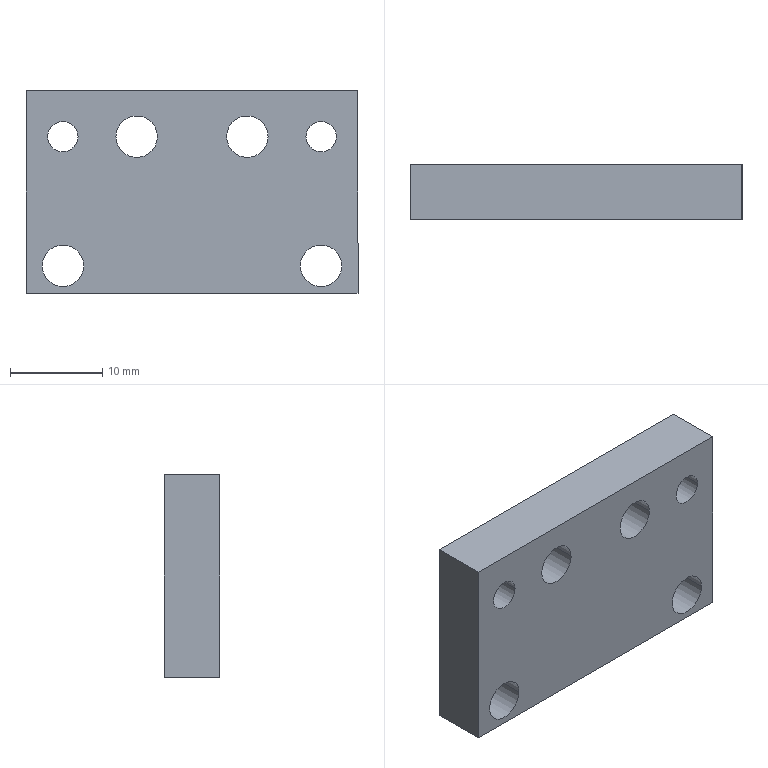Component | SolidWorks | AdjustingPlate-1 | 1 solid | 18 faces | box 36 x 6 x 22 mm | volume 4268 mm3 | cylinder 12 | plane 6 | commonest cylinder face diameters 4.5 x8 3.3 x4
build123d program:
from build123d import *

# Parameters (mm, degrees)
SKETCH1_W                      = 36
SKETCH1_H                      = 22
EXTRUDE1_DEPTH                 = 6
F_4_5_4_5_DIAMETER_HOLE1_D     = 4.5
F_4_5_4_5_DIAMETER_HOLE1_DEPTH = 6.5
F_4_5_4_5_DIAMETER_HOLE1_TIP   = 1.352
SKETCH4_R                      = 2.25
EXTRUDE2_DEPTH                 = 22.932
M4_TAPPED_HOLE1_D              = 3.3
M4_TAPPED_HOLE1_DEPTH          = 11.5
M4_TAPPED_HOLE1_TIP            = 0.9914


with BuildPart() as part:
    # Sketch1 → Extrude1 (new body)
    with BuildSketch(Plane.XY):
        Rectangle(SKETCH1_W, SKETCH1_H)
    extrude(amount=EXTRUDE1_DEPTH)

    # 4.5 _4.5_ Diameter Hole1
    with Locations(Plane.XY.offset(6)):
        with Locations((-14, -8), (14, -8)):
            Hole(F_4_5_4_5_DIAMETER_HOLE1_D / 2, depth=F_4_5_4_5_DIAMETER_HOLE1_DEPTH)
            with Locations((0, 0, -(F_4_5_4_5_DIAMETER_HOLE1_DEPTH + F_4_5_4_5_DIAMETER_HOLE1_TIP / 2))):  # 118° drill point
                Cone(0, F_4_5_4_5_DIAMETER_HOLE1_D / 2, F_4_5_4_5_DIAMETER_HOLE1_TIP, mode=Mode.SUBTRACT)

    # Sketch4 → Extrude2 (cut, through all)
    with BuildSketch(Plane.XY.offset(6)):
        with Locations((-6, 6)):
            Circle(SKETCH4_R)
        with Locations((6, 6)):
            Circle(SKETCH4_R)
    extrude(amount=-EXTRUDE2_DEPTH, mode=Mode.SUBTRACT)

    # M4 Tapped Hole1
    with Locations(Plane.XY.offset(6)):
        with Locations((-14, 6), (14, 6)):
            Hole(M4_TAPPED_HOLE1_D / 2, depth=M4_TAPPED_HOLE1_DEPTH)
            with Locations((0, 0, -(M4_TAPPED_HOLE1_DEPTH + M4_TAPPED_HOLE1_TIP / 2))):  # 118° drill point
                Cone(0, M4_TAPPED_HOLE1_D / 2, M4_TAPPED_HOLE1_TIP, mode=Mode.SUBTRACT)


solid = part.part

# Placed as in the assembly
solid = solid.moved(Location((-50, 166.5, -159.197), (90, 0, 0)))
STEP:
#1=COLOUR_RGB('',0.7922,0.8196,0.9333);
#2=FILL_AREA_STYLE_COLOUR('',#1);
#3=FILL_AREA_STYLE('',(#2));
#4=SURFACE_STYLE_FILL_AREA(#3);
#5=SURFACE_SIDE_STYLE('',(#4));
#6=SURFACE_STYLE_USAGE(.BOTH.,#5);
#7=PRESENTATION_STYLE_ASSIGNMENT((#6));
#8=CARTESIAN_POINT('',(-2.585,6.555,-6.031));
#9=VERTEX_POINT('',#8);
#10=CARTESIAN_POINT('',(-2.455,6.555,-6.031));
#11=VERTEX_POINT('',#10);
#12=CARTESIAN_POINT('',(-2.52,6.555,-6.031));
#13=DIRECTION('',(-0.,-1.,0.));
#14=DIRECTION('',(1.,0.,0.));
#15=AXIS2_PLACEMENT_3D('',#12,#13,#14);
#16=CIRCLE('',#15,0.06496);
#17=EDGE_CURVE('',#9,#11,#16,.T.);
#18=ORIENTED_EDGE('',*,*,#17,.F.);
#19=CARTESIAN_POINT('',(-2.585,6.319,-6.031));
#20=VERTEX_POINT('',#19);
#21=CARTESIAN_POINT('',(-2.585,6.319,-6.031));
#22=DIRECTION('',(-0.,-1.,0.));
#23=VECTOR('',#22,39.37);
#24=LINE('',#21,#23);
#25=EDGE_CURVE('',#9,#20,#24,.T.);
#26=ORIENTED_EDGE('',*,*,#25,.T.);
#27=CARTESIAN_POINT('',(-2.455,6.319,-6.031));
#28=VERTEX_POINT('',#27);
#29=CARTESIAN_POINT('',(-2.52,6.319,-6.031));
#30=DIRECTION('',(-0.,-1.,0.));
#31=DIRECTION('',(1.,0.,0.));
#32=AXIS2_PLACEMENT_3D('',#29,#30,#31);
#33=CIRCLE('',#32,0.06496);
#34=EDGE_CURVE('',#20,#28,#33,.T.);
#35=ORIENTED_EDGE('',*,*,#34,.T.);
#36=CARTESIAN_POINT('',(-2.455,6.319,-6.031));
#37=DIRECTION('',(-0.,-1.,0.));
#38=VECTOR('',#37,39.37);
#39=LINE('',#36,#38);
#40=EDGE_CURVE('',#11,#28,#39,.T.);
#41=ORIENTED_EDGE('',*,*,#40,.F.);
#42=EDGE_LOOP('',(#18,#26,#35,#41));
#43=FACE_OUTER_BOUND('',#42,.T.);
#44=CARTESIAN_POINT('',(-2.52,6.319,-6.031));
#45=DIRECTION('',(-0.,-1.,0.));
#46=DIRECTION('',(1.,0.,0.));
#47=AXIS2_PLACEMENT_3D('',#44,#45,#46);
#48=CYLINDRICAL_SURFACE('',#47,0.06496);
#49=ADVANCED_FACE('',(#43),#48,.F.);
#50=CARTESIAN_POINT('',(-1.482,6.555,-6.031));
#51=VERTEX_POINT('',#50);
#52=CARTESIAN_POINT('',(-1.352,6.555,-6.031));
#53=VERTEX_POINT('',#52);
#54=CARTESIAN_POINT('',(-1.417,6.555,-6.031));
#55=DIRECTION('',(-0.,-1.,0.));
#56=DIRECTION('',(1.,0.,0.));
#57=AXIS2_PLACEMENT_3D('',#54,#55,#56);
#58=CIRCLE('',#57,0.06496);
#59=EDGE_CURVE('',#51,#53,#58,.T.);
#60=ORIENTED_EDGE('',*,*,#59,.F.);
#61=CARTESIAN_POINT('',(-1.482,6.319,-6.031));
#62=VERTEX_POINT('',#61);
#63=CARTESIAN_POINT('',(-1.482,6.319,-6.031));
#64=DIRECTION('',(-0.,-1.,0.));
#65=VECTOR('',#64,39.37);
#66=LINE('',#63,#65);
#67=EDGE_CURVE('',#51,#62,#66,.T.);
#68=ORIENTED_EDGE('',*,*,#67,.T.);
#69=CARTESIAN_POINT('',(-1.352,6.319,-6.031));
#70=VERTEX_POINT('',#69);
#71=CARTESIAN_POINT('',(-1.417,6.319,-6.031));
#72=DIRECTION('',(-0.,-1.,0.));
#73=DIRECTION('',(1.,0.,0.));
#74=AXIS2_PLACEMENT_3D('',#71,#72,#73);
#75=CIRCLE('',#74,0.06496);
#76=EDGE_CURVE('',#62,#70,#75,.T.);
#77=ORIENTED_EDGE('',*,*,#76,.T.);
#78=CARTESIAN_POINT('',(-1.352,6.319,-6.031));
#79=DIRECTION('',(-0.,-1.,0.));
#80=VECTOR('',#79,39.37);
#81=LINE('',#78,#80);
#82=EDGE_CURVE('',#53,#70,#81,.T.);
#83=ORIENTED_EDGE('',*,*,#82,.F.);
#84=EDGE_LOOP('',(#60,#68,#77,#83));
#85=FACE_OUTER_BOUND('',#84,.T.);
#86=CARTESIAN_POINT('',(-1.417,6.319,-6.031));
#87=DIRECTION('',(-0.,-1.,0.));
#88=DIRECTION('',(1.,0.,0.));
#89=AXIS2_PLACEMENT_3D('',#86,#87,#88);
#90=CYLINDRICAL_SURFACE('',#89,0.06496);
#91=ADVANCED_FACE('',(#85),#90,.F.);
#92=CARTESIAN_POINT('',(-1.821,6.555,-6.031));
#93=VERTEX_POINT('',#92);
#94=CARTESIAN_POINT('',(-1.644,6.555,-6.031));
#95=VERTEX_POINT('',#94);
#96=CARTESIAN_POINT('',(-1.732,6.555,-6.031));
#97=DIRECTION('',(-0.,-1.,0.));
#98=DIRECTION('',(1.,0.,0.));
#99=AXIS2_PLACEMENT_3D('',#96,#97,#98);
#100=CIRCLE('',#99,0.08858);
#101=EDGE_CURVE('',#93,#95,#100,.T.);
#102=ORIENTED_EDGE('',*,*,#101,.F.);
#103=CARTESIAN_POINT('',(-1.821,6.319,-6.031));
#104=VERTEX_POINT('',#103);
#105=CARTESIAN_POINT('',(-1.821,6.555,-6.031));
#106=DIRECTION('',(-0.,-1.,0.));
#107=VECTOR('',#106,39.37);
#108=LINE('',#105,#107);
#109=EDGE_CURVE('',#93,#104,#108,.T.);
#110=ORIENTED_EDGE('',*,*,#109,.T.);
#111=CARTESIAN_POINT('',(-1.644,6.319,-6.031));
#112=VERTEX_POINT('',#111);
#113=CARTESIAN_POINT('',(-1.732,6.319,-6.031));
#114=DIRECTION('',(-0.,-1.,0.));
#115=DIRECTION('',(1.,0.,0.));
#116=AXIS2_PLACEMENT_3D('',#113,#114,#115);
#117=CIRCLE('',#116,0.08858);
#118=EDGE_CURVE('',#104,#112,#117,.T.);
#119=ORIENTED_EDGE('',*,*,#118,.T.);
#120=CARTESIAN_POINT('',(-1.644,6.555,-6.031));
#121=DIRECTION('',(-0.,-1.,0.));
#122=VECTOR('',#121,39.37);
#123=LINE('',#120,#122);
#124=EDGE_CURVE('',#95,#112,#123,.T.);
#125=ORIENTED_EDGE('',*,*,#124,.F.);
#126=EDGE_LOOP('',(#102,#110,#119,#125));
#127=FACE_OUTER_BOUND('',#126,.T.);
#128=CARTESIAN_POINT('',(-1.732,6.555,-6.031));
#129=DIRECTION('',(-0.,-1.,0.));
#130=DIRECTION('',(1.,0.,0.));
#131=AXIS2_PLACEMENT_3D('',#128,#129,#130);
#132=CYLINDRICAL_SURFACE('',#131,0.08858);
#133=ADVANCED_FACE('',(#127),#132,.F.);
#134=CARTESIAN_POINT('',(-2.293,6.555,-6.031));
#135=VERTEX_POINT('',#134);
#136=CARTESIAN_POINT('',(-2.116,6.555,-6.031));
#137=VERTEX_POINT('',#136);
#138=CARTESIAN_POINT('',(-2.205,6.555,-6.031));
#139=DIRECTION('',(-0.,-1.,0.));
#140=DIRECTION('',(1.,0.,0.));
#141=AXIS2_PLACEMENT_3D('',#138,#139,#140);
#142=CIRCLE('',#141,0.08858);
#143=EDGE_CURVE('',#135,#137,#142,.T.);
#144=ORIENTED_EDGE('',*,*,#143,.F.);
#145=CARTESIAN_POINT('',(-2.293,6.319,-6.031));
#146=VERTEX_POINT('',#145);
#147=CARTESIAN_POINT('',(-2.293,6.555,-6.031));
#148=DIRECTION('',(-0.,-1.,0.));
#149=VECTOR('',#148,39.37);
#150=LINE('',#147,#149);
#151=EDGE_CURVE('',#135,#146,#150,.T.);
#152=ORIENTED_EDGE('',*,*,#151,.T.);
#153=CARTESIAN_POINT('',(-2.116,6.319,-6.031));
#154=VERTEX_POINT('',#153);
#155=CARTESIAN_POINT('',(-2.205,6.319,-6.031));
#156=DIRECTION('',(-0.,-1.,0.));
#157=DIRECTION('',(1.,0.,0.));
#158=AXIS2_PLACEMENT_3D('',#155,#156,#157);
#159=CIRCLE('',#158,0.08858);
#160=EDGE_CURVE('',#146,#154,#159,.T.);
#161=ORIENTED_EDGE('',*,*,#160,.T.);
#162=CARTESIAN_POINT('',(-2.116,6.555,-6.031));
#163=DIRECTION('',(-0.,-1.,0.));
#164=VECTOR('',#163,39.37);
#165=LINE('',#162,#164);
#166=EDGE_CURVE('',#137,#154,#165,.T.);
#167=ORIENTED_EDGE('',*,*,#166,.F.);
#168=EDGE_LOOP('',(#144,#152,#161,#167));
#169=FACE_OUTER_BOUND('',#168,.T.);
#170=CARTESIAN_POINT('',(-2.205,6.555,-6.031));
#171=DIRECTION('',(-0.,-1.,0.));
#172=DIRECTION('',(1.,0.,0.));
#173=AXIS2_PLACEMENT_3D('',#170,#171,#172);
#174=CYLINDRICAL_SURFACE('',#173,0.08858);
#175=ADVANCED_FACE('',(#169),#174,.F.);
#176=CARTESIAN_POINT('',(-2.608,6.555,-6.583));
#177=VERTEX_POINT('',#176);
#178=CARTESIAN_POINT('',(-2.431,6.555,-6.583));
#179=VERTEX_POINT('',#178);
#180=CARTESIAN_POINT('',(-2.52,6.555,-6.583));
#181=DIRECTION('',(-0.,-1.,0.));
#182=DIRECTION('',(1.,0.,0.));
#183=AXIS2_PLACEMENT_3D('',#180,#181,#182);
#184=CIRCLE('',#183,0.08858);
#185=EDGE_CURVE('',#177,#179,#184,.T.);
#186=ORIENTED_EDGE('',*,*,#185,.F.);
#187=CARTESIAN_POINT('',(-2.608,6.319,-6.583));
#188=VERTEX_POINT('',#187);
#189=CARTESIAN_POINT('',(-2.608,6.319,-6.583));
#190=DIRECTION('',(-0.,-1.,0.));
#191=VECTOR('',#190,39.37);
#192=LINE('',#189,#191);
#193=EDGE_CURVE('',#177,#188,#192,.T.);
#194=ORIENTED_EDGE('',*,*,#193,.T.);
#195=CARTESIAN_POINT('',(-2.431,6.319,-6.583));
#196=VERTEX_POINT('',#195);
#197=CARTESIAN_POINT('',(-2.52,6.319,-6.583));
#198=DIRECTION('',(-0.,-1.,0.));
#199=DIRECTION('',(1.,0.,0.));
#200=AXIS2_PLACEMENT_3D('',#197,#198,#199);
#201=CIRCLE('',#200,0.08858);
#202=EDGE_CURVE('',#188,#196,#201,.T.);
#203=ORIENTED_EDGE('',*,*,#202,.T.);
#204=CARTESIAN_POINT('',(-2.431,6.319,-6.583));
#205=DIRECTION('',(-0.,-1.,0.));
#206=VECTOR('',#205,39.37);
#207=LINE('',#204,#206);
#208=EDGE_CURVE('',#179,#196,#207,.T.);
#209=ORIENTED_EDGE('',*,*,#208,.F.);
#210=EDGE_LOOP('',(#186,#194,#203,#209));
#211=FACE_OUTER_BOUND('',#210,.T.);
#212=CARTESIAN_POINT('',(-2.52,6.319,-6.583));
#213=DIRECTION('',(-0.,-1.,0.));
#214=DIRECTION('',(1.,0.,0.));
#215=AXIS2_PLACEMENT_3D('',#212,#213,#214);
#216=CYLINDRICAL_SURFACE('',#215,0.08858);
#217=ADVANCED_FACE('',(#211),#216,.F.);
#218=CARTESIAN_POINT('',(-1.506,6.555,-6.583));
#219=VERTEX_POINT('',#218);
#220=CARTESIAN_POINT('',(-1.329,6.555,-6.583));
#221=VERTEX_POINT('',#220);
#222=CARTESIAN_POINT('',(-1.417,6.555,-6.583));
#223=DIRECTION('',(-0.,-1.,0.));
#224=DIRECTION('',(1.,0.,0.));
#225=AXIS2_PLACEMENT_3D('',#222,#223,#224);
#226=CIRCLE('',#225,0.08858);
#227=EDGE_CURVE('',#219,#221,#226,.T.);
#228=ORIENTED_EDGE('',*,*,#227,.F.);
#229=CARTESIAN_POINT('',(-1.506,6.319,-6.583));
#230=VERTEX_POINT('',#229);
#231=CARTESIAN_POINT('',(-1.506,6.319,-6.583));
#232=DIRECTION('',(-0.,-1.,0.));
#233=VECTOR('',#232,39.37);
#234=LINE('',#231,#233);
#235=EDGE_CURVE('',#219,#230,#234,.T.);
#236=ORIENTED_EDGE('',*,*,#235,.T.);
#237=CARTESIAN_POINT('',(-1.329,6.319,-6.583));
#238=VERTEX_POINT('',#237);
#239=CARTESIAN_POINT('',(-1.417,6.319,-6.583));
#240=DIRECTION('',(-0.,-1.,0.));
#241=DIRECTION('',(1.,0.,0.));
#242=AXIS2_PLACEMENT_3D('',#239,#240,#241);
#243=CIRCLE('',#242,0.08858);
#244=EDGE_CURVE('',#230,#238,#243,.T.);
#245=ORIENTED_EDGE('',*,*,#244,.T.);
#246=CARTESIAN_POINT('',(-1.329,6.319,-6.583));
#247=DIRECTION('',(-0.,-1.,0.));
#248=VECTOR('',#247,39.37);
#249=LINE('',#246,#248);
#250=EDGE_CURVE('',#221,#238,#249,.T.);
#251=ORIENTED_EDGE('',*,*,#250,.F.);
#252=EDGE_LOOP('',(#228,#236,#245,#251));
#253=FACE_OUTER_BOUND('',#252,.T.);
#254=CARTESIAN_POINT('',(-1.417,6.319,-6.583));
#255=DIRECTION('',(-0.,-1.,0.));
#256=DIRECTION('',(1.,0.,0.));
#257=AXIS2_PLACEMENT_3D('',#254,#255,#256);
#258=CYLINDRICAL_SURFACE('',#257,0.08858);
#259=ADVANCED_FACE('',(#253),#258,.F.);
#260=CARTESIAN_POINT('',(-2.677,6.555,-5.835));
#261=VERTEX_POINT('',#260);
#262=CARTESIAN_POINT('',(-2.677,6.555,-6.701));
#263=VERTEX_POINT('',#262);
#264=CARTESIAN_POINT('',(-2.677,6.555,-6.701));
#265=DIRECTION('',(0.,-0.,-1.));
#266=VECTOR('',#265,39.37);
#267=LINE('',#264,#266);
#268=EDGE_CURVE('',#261,#263,#267,.T.);
#269=ORIENTED_EDGE('',*,*,#268,.T.);
#270=CARTESIAN_POINT('',(-2.677,6.319,-6.701));
#271=VERTEX_POINT('',#270);
#272=CARTESIAN_POINT('',(-2.677,6.319,-6.701));
#273=DIRECTION('',(0.,1.,-0.));
#274=VECTOR('',#273,39.37);
#275=LINE('',#272,#274);
#276=EDGE_CURVE('',#271,#263,#275,.T.);
#277=ORIENTED_EDGE('',*,*,#276,.F.);
#278=CARTESIAN_POINT('',(-2.677,6.319,-5.835));
#279=VERTEX_POINT('',#278);
#280=CARTESIAN_POINT('',(-2.677,6.319,-6.701));
#281=DIRECTION('',(0.,-0.,-1.));
#282=VECTOR('',#281,39.37);
#283=LINE('',#280,#282);
#284=EDGE_CURVE('',#279,#271,#283,.T.);
#285=ORIENTED_EDGE('',*,*,#284,.F.);
#286=CARTESIAN_POINT('',(-2.677,6.319,-5.835));
#287=DIRECTION('',(0.,1.,-0.));
#288=VECTOR('',#287,39.37);
#289=LINE('',#286,#288);
#290=EDGE_CURVE('',#279,#261,#289,.T.);
#291=ORIENTED_EDGE('',*,*,#290,.T.);
#292=EDGE_LOOP('',(#269,#277,#285,#291));
#293=FACE_OUTER_BOUND('',#292,.T.);
#294=CARTESIAN_POINT('',(-2.677,6.319,-6.701));
#295=DIRECTION('',(1.,-0.,0.));
#296=DIRECTION('',(0.,1.,-0.));
#297=AXIS2_PLACEMENT_3D('',#294,#295,#296);
#298=PLANE('',#297);
#299=ADVANCED_FACE('',(#293),#298,.F.);
#300=CARTESIAN_POINT('',(-1.26,6.555,-6.701));
#301=VERTEX_POINT('',#300);
#302=CARTESIAN_POINT('',(-1.26,6.555,-6.701));
#303=DIRECTION('',(1.,-0.,0.));
#304=VECTOR('',#303,39.37);
#305=LINE('',#302,#304);
#306=EDGE_CURVE('',#263,#301,#305,.T.);
#307=ORIENTED_EDGE('',*,*,#306,.T.);
#308=CARTESIAN_POINT('',(-1.26,6.319,-6.701));
#309=VERTEX_POINT('',#308);
#310=CARTESIAN_POINT('',(-1.26,6.319,-6.701));
#311=DIRECTION('',(0.,1.,-0.));
#312=VECTOR('',#311,39.37);
#313=LINE('',#310,#312);
#314=EDGE_CURVE('',#309,#301,#313,.T.);
#315=ORIENTED_EDGE('',*,*,#314,.F.);
#316=CARTESIAN_POINT('',(-1.26,6.319,-6.701));
#317=DIRECTION('',(1.,-0.,0.));
#318=VECTOR('',#317,39.37);
#319=LINE('',#316,#318);
#320=EDGE_CURVE('',#271,#309,#319,.T.);
#321=ORIENTED_EDGE('',*,*,#320,.F.);
#322=ORIENTED_EDGE('',*,*,#276,.T.);
#323=EDGE_LOOP('',(#307,#315,#321,#322));
#324=FACE_OUTER_BOUND('',#323,.T.);
#325=CARTESIAN_POINT('',(-1.26,6.319,-6.701));
#326=DIRECTION('',(-0.,0.,1.));
#327=DIRECTION('',(-1.,0.,-0.));
#328=AXIS2_PLACEMENT_3D('',#325,#326,#327);
#329=PLANE('',#328);
#330=ADVANCED_FACE('',(#324),#329,.F.);
#331=CARTESIAN_POINT('',(-1.26,6.555,-5.835));
#332=VERTEX_POINT('',#331);
#333=CARTESIAN_POINT('',(-1.26,6.555,-6.701));
#334=DIRECTION('',(-0.,0.,1.));
#335=VECTOR('',#334,39.37);
#336=LINE('',#333,#335);
#337=EDGE_CURVE('',#301,#332,#336,.T.);
#338=ORIENTED_EDGE('',*,*,#337,.T.);
#339=CARTESIAN_POINT('',(-1.26,6.319,-5.835));
#340=VERTEX_POINT('',#339);
#341=CARTESIAN_POINT('',(-1.26,6.319,-5.835));
#342=DIRECTION('',(0.,1.,-0.));
#343=VECTOR('',#342,39.37);
#344=LINE('',#341,#343);
#345=EDGE_CURVE('',#340,#332,#344,.T.);
#346=ORIENTED_EDGE('',*,*,#345,.F.);
#347=CARTESIAN_POINT('',(-1.26,6.319,-6.701));
#348=DIRECTION('',(-0.,0.,1.));
#349=VECTOR('',#348,39.37);
#350=LINE('',#347,#349);
#351=EDGE_CURVE('',#309,#340,#350,.T.);
#352=ORIENTED_EDGE('',*,*,#351,.F.);
#353=ORIENTED_EDGE('',*,*,#314,.T.);
#354=EDGE_LOOP('',(#338,#346,#352,#353));
#355=FACE_OUTER_BOUND('',#354,.T.);
#356=CARTESIAN_POINT('',(-1.26,6.319,-6.701));
#357=DIRECTION('',(-1.,0.,-0.));
#358=DIRECTION('',(-0.,-1.,0.));
#359=AXIS2_PLACEMENT_3D('',#356,#357,#358);
#360=PLANE('',#359);
#361=ADVANCED_FACE('',(#355),#360,.F.);
#362=CARTESIAN_POINT('',(-1.26,6.555,-5.835));
#363=DIRECTION('',(-1.,0.,-0.));
#364=VECTOR('',#363,39.37);
#365=LINE('',#362,#364);
#366=EDGE_CURVE('',#332,#261,#365,.T.);
#367=ORIENTED_EDGE('',*,*,#366,.T.);
#368=ORIENTED_EDGE('',*,*,#290,.F.);
#369=CARTESIAN_POINT('',(-1.26,6.319,-5.835));
#370=DIRECTION('',(-1.,0.,-0.));
#371=VECTOR('',#370,39.37);
#372=LINE('',#369,#371);
#373=EDGE_CURVE('',#340,#279,#372,.T.);
#374=ORIENTED_EDGE('',*,*,#373,.F.);
#375=ORIENTED_EDGE('',*,*,#345,.T.);
#376=EDGE_LOOP('',(#367,#368,#374,#375));
#377=FACE_OUTER_BOUND('',#376,.T.);
#378=CARTESIAN_POINT('',(-1.26,6.319,-5.835));
#379=DIRECTION('',(0.,-0.,-1.));
#380=DIRECTION('',(1.,-0.,0.));
#381=AXIS2_PLACEMENT_3D('',#378,#379,#380);
#382=PLANE('',#381);
#383=ADVANCED_FACE('',(#377),#382,.F.);
#384=CARTESIAN_POINT('',(-2.52,6.319,-6.031));
#385=DIRECTION('',(-0.,-1.,0.));
#386=DIRECTION('',(1.,0.,0.));
#387=AXIS2_PLACEMENT_3D('',#384,#385,#386);
#388=CIRCLE('',#387,0.06496);
#389=EDGE_CURVE('',#28,#20,#388,.T.);
#390=ORIENTED_EDGE('',*,*,#389,.F.);
#391=ORIENTED_EDGE('',*,*,#34,.F.);
#392=EDGE_LOOP('',(#390,#391));
#393=FACE_BOUND('',#392,.T.);
#394=CARTESIAN_POINT('',(-1.417,6.319,-6.031));
#395=DIRECTION('',(-0.,-1.,0.));
#396=DIRECTION('',(1.,0.,0.));
#397=AXIS2_PLACEMENT_3D('',#394,#395,#396);
#398=CIRCLE('',#397,0.06496);
#399=EDGE_CURVE('',#70,#62,#398,.T.);
#400=ORIENTED_EDGE('',*,*,#399,.F.);
#401=ORIENTED_EDGE('',*,*,#76,.F.);
#402=EDGE_LOOP('',(#400,#401));
#403=FACE_BOUND('',#402,.T.);
#404=CARTESIAN_POINT('',(-1.732,6.319,-6.031));
#405=DIRECTION('',(-0.,-1.,0.));
#406=DIRECTION('',(1.,0.,0.));
#407=AXIS2_PLACEMENT_3D('',#404,#405,#406);
#408=CIRCLE('',#407,0.08858);
#409=EDGE_CURVE('',#112,#104,#408,.T.);
#410=ORIENTED_EDGE('',*,*,#409,.F.);
#411=ORIENTED_EDGE('',*,*,#118,.F.);
#412=EDGE_LOOP('',(#410,#411));
#413=FACE_BOUND('',#412,.T.);
#414=CARTESIAN_POINT('',(-2.205,6.319,-6.031));
#415=DIRECTION('',(-0.,-1.,0.));
#416=DIRECTION('',(1.,0.,0.));
#417=AXIS2_PLACEMENT_3D('',#414,#415,#416);
#418=CIRCLE('',#417,0.08858);
#419=EDGE_CURVE('',#154,#146,#418,.T.);
#420=ORIENTED_EDGE('',*,*,#419,.F.);
#421=ORIENTED_EDGE('',*,*,#160,.F.);
#422=EDGE_LOOP('',(#420,#421));
#423=FACE_BOUND('',#422,.T.);
#424=CARTESIAN_POINT('',(-2.52,6.319,-6.583));
#425=DIRECTION('',(-0.,-1.,0.));
#426=DIRECTION('',(1.,0.,0.));
#427=AXIS2_PLACEMENT_3D('',#424,#425,#426);
#428=CIRCLE('',#427,0.08858);
#429=EDGE_CURVE('',#196,#188,#428,.T.);
#430=ORIENTED_EDGE('',*,*,#429,.F.);
#431=ORIENTED_EDGE('',*,*,#202,.F.);
#432=EDGE_LOOP('',(#430,#431));
#433=FACE_BOUND('',#432,.T.);
#434=CARTESIAN_POINT('',(-1.417,6.319,-6.583));
#435=DIRECTION('',(-0.,-1.,0.));
#436=DIRECTION('',(1.,0.,0.));
#437=AXIS2_PLACEMENT_3D('',#434,#435,#436);
#438=CIRCLE('',#437,0.08858);
#439=EDGE_CURVE('',#238,#230,#438,.T.);
#440=ORIENTED_EDGE('',*,*,#439,.F.);
#441=ORIENTED_EDGE('',*,*,#244,.F.);
#442=EDGE_LOOP('',(#440,#441));
#443=FACE_BOUND('',#442,.T.);
#444=ORIENTED_EDGE('',*,*,#284,.T.);
#445=ORIENTED_EDGE('',*,*,#320,.T.);
#446=ORIENTED_EDGE('',*,*,#351,.T.);
#447=ORIENTED_EDGE('',*,*,#373,.T.);
#448=EDGE_LOOP('',(#444,#445,#446,#447));
#449=FACE_OUTER_BOUND('',#448,.T.);
#450=CARTESIAN_POINT('',(-2.677,6.319,-5.835));
#451=DIRECTION('',(-0.,-1.,0.));
#452=DIRECTION('',(1.,-0.,0.));
#453=AXIS2_PLACEMENT_3D('',#450,#451,#452);
#454=PLANE('',#453);
#455=ADVANCED_FACE('',(#393,#403,#413,#423,#433,#443,#449),#454,.T.);
#456=CARTESIAN_POINT('',(-2.52,6.555,-6.031));
#457=DIRECTION('',(-0.,-1.,0.));
#458=DIRECTION('',(1.,0.,0.));
#459=AXIS2_PLACEMENT_3D('',#456,#457,#458);
#460=CIRCLE('',#459,0.06496);
#461=EDGE_CURVE('',#11,#9,#460,.T.);
#462=ORIENTED_EDGE('',*,*,#461,.T.);
#463=ORIENTED_EDGE('',*,*,#17,.T.);
#464=EDGE_LOOP('',(#462,#463));
#465=FACE_BOUND('',#464,.T.);
#466=CARTESIAN_POINT('',(-1.417,6.555,-6.031));
#467=DIRECTION('',(-0.,-1.,0.));
#468=DIRECTION('',(1.,0.,0.));
#469=AXIS2_PLACEMENT_3D('',#466,#467,#468);
#470=CIRCLE('',#469,0.06496);
#471=EDGE_CURVE('',#53,#51,#470,.T.);
#472=ORIENTED_EDGE('',*,*,#471,.T.);
#473=ORIENTED_EDGE('',*,*,#59,.T.);
#474=EDGE_LOOP('',(#472,#473));
#475=FACE_BOUND('',#474,.T.);
#476=CARTESIAN_POINT('',(-1.732,6.555,-6.031));
#477=DIRECTION('',(-0.,-1.,0.));
#478=DIRECTION('',(1.,0.,0.));
#479=AXIS2_PLACEMENT_3D('',#476,#477,#478);
#480=CIRCLE('',#479,0.08858);
#481=EDGE_CURVE('',#95,#93,#480,.T.);
#482=ORIENTED_EDGE('',*,*,#481,.T.);
#483=ORIENTED_EDGE('',*,*,#101,.T.);
#484=EDGE_LOOP('',(#482,#483));
#485=FACE_BOUND('',#484,.T.);
#486=CARTESIAN_POINT('',(-2.205,6.555,-6.031));
#487=DIRECTION('',(-0.,-1.,0.));
#488=DIRECTION('',(1.,0.,0.));
#489=AXIS2_PLACEMENT_3D('',#486,#487,#488);
#490=CIRCLE('',#489,0.08858);
#491=EDGE_CURVE('',#137,#135,#490,.T.);
#492=ORIENTED_EDGE('',*,*,#491,.T.);
#493=ORIENTED_EDGE('',*,*,#143,.T.);
#494=EDGE_LOOP('',(#492,#493));
#495=FACE_BOUND('',#494,.T.);
#496=CARTESIAN_POINT('',(-2.52,6.555,-6.583));
#497=DIRECTION('',(-0.,-1.,0.));
#498=DIRECTION('',(1.,0.,0.));
#499=AXIS2_PLACEMENT_3D('',#496,#497,#498);
#500=CIRCLE('',#499,0.08858);
#501=EDGE_CURVE('',#179,#177,#500,.T.);
#502=ORIENTED_EDGE('',*,*,#501,.T.);
#503=ORIENTED_EDGE('',*,*,#185,.T.);
#504=EDGE_LOOP('',(#502,#503));
#505=FACE_BOUND('',#504,.T.);
#506=CARTESIAN_POINT('',(-1.417,6.555,-6.583));
#507=DIRECTION('',(-0.,-1.,0.));
#508=DIRECTION('',(1.,0.,0.));
#509=AXIS2_PLACEMENT_3D('',#506,#507,#508);
#510=CIRCLE('',#509,0.08858);
#511=EDGE_CURVE('',#221,#219,#510,.T.);
#512=ORIENTED_EDGE('',*,*,#511,.T.);
#513=ORIENTED_EDGE('',*,*,#227,.T.);
#514=EDGE_LOOP('',(#512,#513));
#515=FACE_BOUND('',#514,.T.);
#516=ORIENTED_EDGE('',*,*,#268,.F.);
#517=ORIENTED_EDGE('',*,*,#366,.F.);
#518=ORIENTED_EDGE('',*,*,#337,.F.);
#519=ORIENTED_EDGE('',*,*,#306,.F.);
#520=EDGE_LOOP('',(#516,#517,#518,#519));
#521=FACE_OUTER_BOUND('',#520,.T.);
#522=CARTESIAN_POINT('',(-2.677,6.555,-5.835));
#523=DIRECTION('',(-0.,-1.,0.));
#524=DIRECTION('',(1.,-0.,0.));
#525=AXIS2_PLACEMENT_3D('',#522,#523,#524);
#526=PLANE('',#525);
#527=ADVANCED_FACE('',(#465,#475,#485,#495,#505,#515,#521),#526,.F.);
#528=ORIENTED_EDGE('',*,*,#235,.F.);
#529=ORIENTED_EDGE('',*,*,#511,.F.);
#530=ORIENTED_EDGE('',*,*,#250,.T.);
#531=ORIENTED_EDGE('',*,*,#439,.T.);
#532=EDGE_LOOP('',(#528,#529,#530,#531));
#533=FACE_OUTER_BOUND('',#532,.T.);
#534=CARTESIAN_POINT('',(-1.417,6.319,-6.583));
#535=DIRECTION('',(-0.,-1.,0.));
#536=DIRECTION('',(1.,0.,0.));
#537=AXIS2_PLACEMENT_3D('',#534,#535,#536);
#538=CYLINDRICAL_SURFACE('',#537,0.08858);
#539=ADVANCED_FACE('',(#533),#538,.F.);
#540=ORIENTED_EDGE('',*,*,#193,.F.);
#541=ORIENTED_EDGE('',*,*,#501,.F.);
#542=ORIENTED_EDGE('',*,*,#208,.T.);
#543=ORIENTED_EDGE('',*,*,#429,.T.);
#544=EDGE_LOOP('',(#540,#541,#542,#543));
#545=FACE_OUTER_BOUND('',#544,.T.);
#546=CARTESIAN_POINT('',(-2.52,6.319,-6.583));
#547=DIRECTION('',(-0.,-1.,0.));
#548=DIRECTION('',(1.,0.,0.));
#549=AXIS2_PLACEMENT_3D('',#546,#547,#548);
#550=CYLINDRICAL_SURFACE('',#549,0.08858);
#551=ADVANCED_FACE('',(#545),#550,.F.);
#552=ORIENTED_EDGE('',*,*,#151,.F.);
#553=ORIENTED_EDGE('',*,*,#491,.F.);
#554=ORIENTED_EDGE('',*,*,#166,.T.);
#555=ORIENTED_EDGE('',*,*,#419,.T.);
#556=EDGE_LOOP('',(#552,#553,#554,#555));
#557=FACE_OUTER_BOUND('',#556,.T.);
#558=CARTESIAN_POINT('',(-2.205,6.555,-6.031));
#559=DIRECTION('',(-0.,-1.,0.));
#560=DIRECTION('',(1.,0.,0.));
#561=AXIS2_PLACEMENT_3D('',#558,#559,#560);
#562=CYLINDRICAL_SURFACE('',#561,0.08858);
#563=ADVANCED_FACE('',(#557),#562,.F.);
#564=ORIENTED_EDGE('',*,*,#109,.F.);
#565=ORIENTED_EDGE('',*,*,#481,.F.);
#566=ORIENTED_EDGE('',*,*,#124,.T.);
#567=ORIENTED_EDGE('',*,*,#409,.T.);
#568=EDGE_LOOP('',(#564,#565,#566,#567));
#569=FACE_OUTER_BOUND('',#568,.T.);
#570=CARTESIAN_POINT('',(-1.732,6.555,-6.031));
#571=DIRECTION('',(-0.,-1.,0.));
#572=DIRECTION('',(1.,0.,0.));
#573=AXIS2_PLACEMENT_3D('',#570,#571,#572);
#574=CYLINDRICAL_SURFACE('',#573,0.08858);
#575=ADVANCED_FACE('',(#569),#574,.F.);
#576=ORIENTED_EDGE('',*,*,#67,.F.);
#577=ORIENTED_EDGE('',*,*,#471,.F.);
#578=ORIENTED_EDGE('',*,*,#82,.T.);
#579=ORIENTED_EDGE('',*,*,#399,.T.);
#580=EDGE_LOOP('',(#576,#577,#578,#579));
#581=FACE_OUTER_BOUND('',#580,.T.);
#582=CARTESIAN_POINT('',(-1.417,6.319,-6.031));
#583=DIRECTION('',(-0.,-1.,0.));
#584=DIRECTION('',(1.,0.,0.));
#585=AXIS2_PLACEMENT_3D('',#582,#583,#584);
#586=CYLINDRICAL_SURFACE('',#585,0.06496);
#587=ADVANCED_FACE('',(#581),#586,.F.);
#588=ORIENTED_EDGE('',*,*,#25,.F.);
#589=ORIENTED_EDGE('',*,*,#461,.F.);
#590=ORIENTED_EDGE('',*,*,#40,.T.);
#591=ORIENTED_EDGE('',*,*,#389,.T.);
#592=EDGE_LOOP('',(#588,#589,#590,#591));
#593=FACE_OUTER_BOUND('',#592,.T.);
#594=CARTESIAN_POINT('',(-2.52,6.319,-6.031));
#595=DIRECTION('',(-0.,-1.,0.));
#596=DIRECTION('',(1.,0.,0.));
#597=AXIS2_PLACEMENT_3D('',#594,#595,#596);
#598=CYLINDRICAL_SURFACE('',#597,0.06496);
#599=ADVANCED_FACE('',(#593),#598,.F.);
#600=CLOSED_SHELL('',(#49,#91,#133,#175,#217,#259,#299,#330,#361,#383,#455,#527,#539,#551,#563,#575,#587,#599));
#601=MANIFOLD_SOLID_BREP('',#600);
#602=STYLED_ITEM('',(#7),#601);
#603=(LENGTH_UNIT()NAMED_UNIT(*)SI_UNIT($,.METRE.));
#604=LENGTH_MEASURE_WITH_UNIT(LENGTH_MEASURE(0.0254),#603);
#605=DIMENSIONAL_EXPONENTS(1.,0.,0.,0.,0.,0.,0.);
#606=(CONVERSION_BASED_UNIT('',#604)LENGTH_UNIT()NAMED_UNIT(#605));
#607=UNCERTAINTY_MEASURE_WITH_UNIT(LENGTH_MEASURE(0.00001),#606,'','');
#608=(NAMED_UNIT(*)PLANE_ANGLE_UNIT()SI_UNIT($,.RADIAN.));
#609=(NAMED_UNIT(*)SI_UNIT($,.STERADIAN.)SOLID_ANGLE_UNIT());
#610=(GEOMETRIC_REPRESENTATION_CONTEXT(3)GLOBAL_UNCERTAINTY_ASSIGNED_CONTEXT((#607))GLOBAL_UNIT_ASSIGNED_CONTEXT((#606,#608,#609))REPRESENTATION_CONTEXT('',''));
#611=MECHANICAL_DESIGN_GEOMETRIC_PRESENTATION_REPRESENTATION('',(#602),#610);
#612=CARTESIAN_POINT('',(0.,0.,0.));
#613=DIRECTION('',(0.,0.,1.));
#614=DIRECTION('',(1.,0.,0.));
#615=AXIS2_PLACEMENT_3D('',#612,#613,#614);
#616=(LENGTH_UNIT()NAMED_UNIT(*)SI_UNIT($,.METRE.));
#617=LENGTH_MEASURE_WITH_UNIT(LENGTH_MEASURE(0.0254),#616);
#618=DIMENSIONAL_EXPONENTS(1.,0.,0.,0.,0.,0.,0.);
#619=(CONVERSION_BASED_UNIT('',#617)LENGTH_UNIT()NAMED_UNIT(#618));
#620=UNCERTAINTY_MEASURE_WITH_UNIT(LENGTH_MEASURE(0.00001),#619,'','');
#621=(NAMED_UNIT(*)PLANE_ANGLE_UNIT()SI_UNIT($,.RADIAN.));
#622=(NAMED_UNIT(*)SI_UNIT($,.STERADIAN.)SOLID_ANGLE_UNIT());
#623=(GEOMETRIC_REPRESENTATION_CONTEXT(3)GLOBAL_UNCERTAINTY_ASSIGNED_CONTEXT((#620))GLOBAL_UNIT_ASSIGNED_CONTEXT((#619,#621,#622))REPRESENTATION_CONTEXT('',''));
#624=ADVANCED_BREP_SHAPE_REPRESENTATION('',(#601,#615),#623);
#625=PRESENTATION_LAYER_ASSIGNMENT('','',(#602));